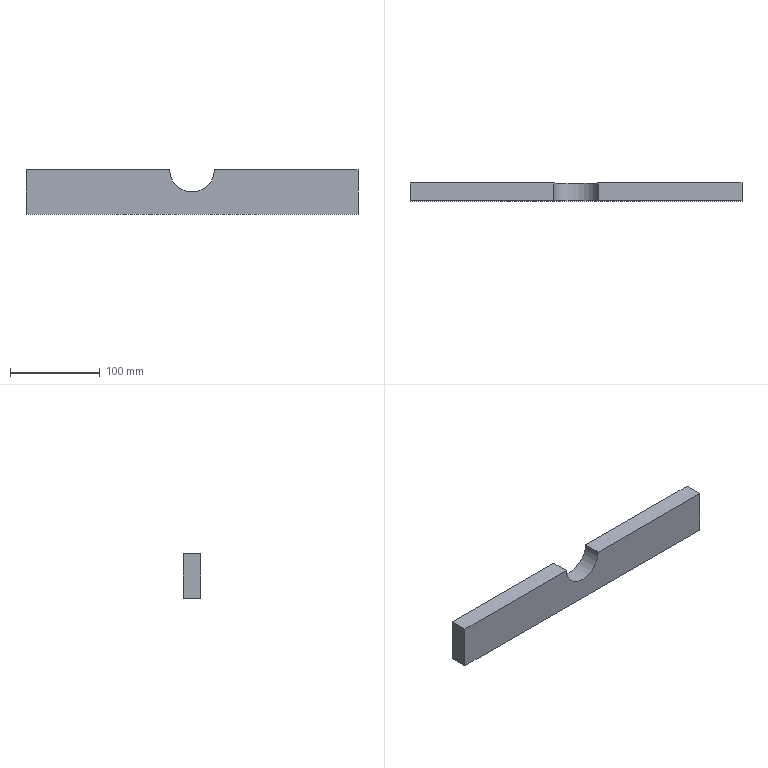Component | NX | TUTUCU_2 | 1 solid | 8 faces | box 370 x 20 x 50 mm | volume 350365 mm3 | plane 7 | cylinder 1 | commonest cylinder face diameters 50 x1
STEP:
#1=CARTESIAN_POINT('',(0.,0.,0.));
#2=DIRECTION('',(0.,0.,1.));
#3=DIRECTION('',(1.,0.,0.));
#4=AXIS2_PLACEMENT_3D('',#1,#2,#3);
#5=CARTESIAN_POINT('',(-1180.866,789.623,220.));
#6=VERTEX_POINT('',#5);
#7=CARTESIAN_POINT('',(-1180.866,769.623,220.));
#8=VERTEX_POINT('',#7);
#9=CARTESIAN_POINT('',(-1180.866,767.623,220.));
#10=DIRECTION('',(0.,-1.,0.));
#11=VECTOR('',#10,1.);
#12=LINE('',#9,#11);
#13=CARTESIAN_POINT('',(-970.866,789.623,220.));
#14=DIRECTION('',(0.,0.,-1.));
#15=DIRECTION('',(-1.,0.,0.));
#16=AXIS2_PLACEMENT_3D('',#13,#14,#15);
#17=PLANE('',#16);
#18=CARTESIAN_POINT('',(210.,-22.));
#19=DIRECTION('',(0.,-1.));
#20=VECTOR('',#19,1.);
#21=LINE('',#18,#20);
#22=(GEOMETRIC_REPRESENTATION_CONTEXT(2)PARAMETRIC_REPRESENTATION_CONTEXT()REPRESENTATION_CONTEXT('',''));
#23=DEFINITIONAL_REPRESENTATION('',(#21),#22);
#24=PCURVE('',#17,#23);
#25=CARTESIAN_POINT('',(-1155.866,767.623,220.));
#26=DIRECTION('',(0.,1.,0.));
#27=DIRECTION('',(0.,0.,1.));
#28=AXIS2_PLACEMENT_3D('',#25,#26,#27);
#29=CYLINDRICAL_SURFACE('',#28,25.);
#30=CARTESIAN_POINT('',(4.712,0.));
#31=DIRECTION('',(0.,-1.));
#32=VECTOR('',#31,1.);
#33=LINE('',#30,#32);
#34=(GEOMETRIC_REPRESENTATION_CONTEXT(2)PARAMETRIC_REPRESENTATION_CONTEXT()REPRESENTATION_CONTEXT('',''));
#35=DEFINITIONAL_REPRESENTATION('',(#33),#34);
#36=PCURVE('',#29,#35);
#37=SURFACE_CURVE('',#12,(#24,#36),.PCURVE_S1.);
#38=EDGE_CURVE('',#6,#8,#37,.T.);
#39=ORIENTED_EDGE('',*,*,#38,.F.);
#40=CARTESIAN_POINT('',(-1340.866,789.623,220.));
#41=VERTEX_POINT('',#40);
#42=CARTESIAN_POINT('',(-970.866,789.623,220.));
#43=DIRECTION('',(-1.,0.,0.));
#44=VECTOR('',#43,1.);
#45=LINE('',#42,#44);
#46=CARTESIAN_POINT('',(0.,0.));
#47=DIRECTION('',(1.,0.));
#48=VECTOR('',#47,1.);
#49=LINE('',#46,#48);
#50=(GEOMETRIC_REPRESENTATION_CONTEXT(2)PARAMETRIC_REPRESENTATION_CONTEXT()REPRESENTATION_CONTEXT('',''));
#51=DEFINITIONAL_REPRESENTATION('',(#49),#50);
#52=PCURVE('',#17,#51);
#53=CARTESIAN_POINT('',(-970.866,789.623,170.));
#54=DIRECTION('',(0.,-1.,-0.));
#55=DIRECTION('',(0.,0.,-1.));
#56=AXIS2_PLACEMENT_3D('',#53,#54,#55);
#57=PLANE('',#56);
#58=CARTESIAN_POINT('',(-50.,0.));
#59=DIRECTION('',(0.,-1.));
#60=VECTOR('',#59,1.);
#61=LINE('',#58,#60);
#62=(GEOMETRIC_REPRESENTATION_CONTEXT(2)PARAMETRIC_REPRESENTATION_CONTEXT()REPRESENTATION_CONTEXT('',''));
#63=DEFINITIONAL_REPRESENTATION('',(#61),#62);
#64=PCURVE('',#57,#63);
#65=SURFACE_CURVE('',#45,(#52,#64),.PCURVE_S1.);
#66=EDGE_CURVE('',#6,#41,#65,.T.);
#67=ORIENTED_EDGE('',*,*,#66,.T.);
#68=CARTESIAN_POINT('',(-1340.866,769.623,220.));
#69=VERTEX_POINT('',#68);
#70=CARTESIAN_POINT('',(-1340.866,789.623,220.));
#71=DIRECTION('',(0.,-1.,0.));
#72=VECTOR('',#71,1.);
#73=LINE('',#70,#72);
#74=CARTESIAN_POINT('',(370.,0.));
#75=DIRECTION('',(0.,-1.));
#76=VECTOR('',#75,1.);
#77=LINE('',#74,#76);
#78=(GEOMETRIC_REPRESENTATION_CONTEXT(2)PARAMETRIC_REPRESENTATION_CONTEXT()REPRESENTATION_CONTEXT('',''));
#79=DEFINITIONAL_REPRESENTATION('',(#77),#78);
#80=PCURVE('',#17,#79);
#81=CARTESIAN_POINT('',(-1340.866,769.623,170.));
#82=DIRECTION('',(1.,0.,0.));
#83=DIRECTION('',(0.,0.,-1.));
#84=AXIS2_PLACEMENT_3D('',#81,#82,#83);
#85=PLANE('',#84);
#86=CARTESIAN_POINT('',(-50.,20.));
#87=DIRECTION('',(0.,-1.));
#88=VECTOR('',#87,1.);
#89=LINE('',#86,#88);
#90=(GEOMETRIC_REPRESENTATION_CONTEXT(2)PARAMETRIC_REPRESENTATION_CONTEXT()REPRESENTATION_CONTEXT('',''));
#91=DEFINITIONAL_REPRESENTATION('',(#89),#90);
#92=PCURVE('',#85,#91);
#93=SURFACE_CURVE('',#73,(#80,#92),.PCURVE_S1.);
#94=EDGE_CURVE('',#41,#69,#93,.T.);
#95=ORIENTED_EDGE('',*,*,#94,.T.);
#96=CARTESIAN_POINT('',(-970.866,769.623,220.));
#97=DIRECTION('',(-1.,0.,0.));
#98=VECTOR('',#97,1.);
#99=LINE('',#96,#98);
#100=CARTESIAN_POINT('',(0.,-20.));
#101=DIRECTION('',(1.,0.));
#102=VECTOR('',#101,1.);
#103=LINE('',#100,#102);
#104=(GEOMETRIC_REPRESENTATION_CONTEXT(2)PARAMETRIC_REPRESENTATION_CONTEXT()REPRESENTATION_CONTEXT('',''));
#105=DEFINITIONAL_REPRESENTATION('',(#103),#104);
#106=PCURVE('',#17,#105);
#107=CARTESIAN_POINT('',(-970.866,769.623,220.));
#108=DIRECTION('',(0.,1.,0.));
#109=DIRECTION('',(0.,-0.,1.));
#110=AXIS2_PLACEMENT_3D('',#107,#108,#109);
#111=PLANE('',#110);
#112=CARTESIAN_POINT('',(0.,0.));
#113=DIRECTION('',(0.,-1.));
#114=VECTOR('',#113,1.);
#115=LINE('',#112,#114);
#116=(GEOMETRIC_REPRESENTATION_CONTEXT(2)PARAMETRIC_REPRESENTATION_CONTEXT()REPRESENTATION_CONTEXT('',''));
#117=DEFINITIONAL_REPRESENTATION('',(#115),#116);
#118=PCURVE('',#111,#117);
#119=SURFACE_CURVE('',#99,(#106,#118),.PCURVE_S1.);
#120=EDGE_CURVE('',#8,#69,#119,.T.);
#121=ORIENTED_EDGE('',*,*,#120,.F.);
#122=EDGE_LOOP('',(#39,#67,#95,#121));
#123=FACE_BOUND('',#122,.T.);
#124=ADVANCED_FACE('',(#123),#17,.F.);
#125=CARTESIAN_POINT('',(-1130.866,769.623,220.));
#126=VERTEX_POINT('',#125);
#127=CARTESIAN_POINT('',(-1130.866,789.623,220.));
#128=VERTEX_POINT('',#127);
#129=CARTESIAN_POINT('',(-1130.866,767.623,220.));
#130=DIRECTION('',(0.,1.,0.));
#131=VECTOR('',#130,1.);
#132=LINE('',#129,#131);
#133=CARTESIAN_POINT('',(-970.866,789.623,220.));
#134=DIRECTION('',(0.,0.,-1.));
#135=DIRECTION('',(-1.,0.,0.));
#136=AXIS2_PLACEMENT_3D('',#133,#134,#135);
#137=PLANE('',#136);
#138=CARTESIAN_POINT('',(160.,-22.));
#139=DIRECTION('',(0.,1.));
#140=VECTOR('',#139,1.);
#141=LINE('',#138,#140);
#142=(GEOMETRIC_REPRESENTATION_CONTEXT(2)PARAMETRIC_REPRESENTATION_CONTEXT()REPRESENTATION_CONTEXT('',''));
#143=DEFINITIONAL_REPRESENTATION('',(#141),#142);
#144=PCURVE('',#137,#143);
#145=CARTESIAN_POINT('',(1.571,0.));
#146=DIRECTION('',(0.,1.));
#147=VECTOR('',#146,1.);
#148=LINE('',#145,#147);
#149=(GEOMETRIC_REPRESENTATION_CONTEXT(2)PARAMETRIC_REPRESENTATION_CONTEXT()REPRESENTATION_CONTEXT('',''));
#150=DEFINITIONAL_REPRESENTATION('',(#148),#149);
#151=PCURVE('',#29,#150);
#152=SURFACE_CURVE('',#132,(#144,#151),.PCURVE_S1.);
#153=EDGE_CURVE('',#126,#128,#152,.T.);
#154=ORIENTED_EDGE('',*,*,#153,.F.);
#155=CARTESIAN_POINT('',(-970.866,769.623,220.));
#156=VERTEX_POINT('',#155);
#157=CARTESIAN_POINT('',(-970.866,769.623,220.));
#158=DIRECTION('',(-1.,0.,0.));
#159=VECTOR('',#158,1.);
#160=LINE('',#157,#159);
#161=CARTESIAN_POINT('',(0.,-20.));
#162=DIRECTION('',(1.,0.));
#163=VECTOR('',#162,1.);
#164=LINE('',#161,#163);
#165=(GEOMETRIC_REPRESENTATION_CONTEXT(2)PARAMETRIC_REPRESENTATION_CONTEXT()REPRESENTATION_CONTEXT('',''));
#166=DEFINITIONAL_REPRESENTATION('',(#164),#165);
#167=PCURVE('',#137,#166);
#168=CARTESIAN_POINT('',(0.,0.));
#169=DIRECTION('',(0.,-1.));
#170=VECTOR('',#169,1.);
#171=LINE('',#168,#170);
#172=(GEOMETRIC_REPRESENTATION_CONTEXT(2)PARAMETRIC_REPRESENTATION_CONTEXT()REPRESENTATION_CONTEXT('',''));
#173=DEFINITIONAL_REPRESENTATION('',(#171),#172);
#174=PCURVE('',#111,#173);
#175=SURFACE_CURVE('',#160,(#167,#174),.PCURVE_S1.);
#176=EDGE_CURVE('',#156,#126,#175,.T.);
#177=ORIENTED_EDGE('',*,*,#176,.F.);
#178=CARTESIAN_POINT('',(-970.866,789.623,220.));
#179=VERTEX_POINT('',#178);
#180=CARTESIAN_POINT('',(-970.866,789.623,220.));
#181=DIRECTION('',(0.,-1.,0.));
#182=VECTOR('',#181,1.);
#183=LINE('',#180,#182);
#184=CARTESIAN_POINT('',(0.,0.));
#185=DIRECTION('',(0.,-1.));
#186=VECTOR('',#185,1.);
#187=LINE('',#184,#186);
#188=(GEOMETRIC_REPRESENTATION_CONTEXT(2)PARAMETRIC_REPRESENTATION_CONTEXT()REPRESENTATION_CONTEXT('',''));
#189=DEFINITIONAL_REPRESENTATION('',(#187),#188);
#190=PCURVE('',#137,#189);
#191=CARTESIAN_POINT('',(-970.866,769.623,170.));
#192=DIRECTION('',(1.,0.,0.));
#193=DIRECTION('',(0.,0.,-1.));
#194=AXIS2_PLACEMENT_3D('',#191,#192,#193);
#195=PLANE('',#194);
#196=CARTESIAN_POINT('',(-50.,20.));
#197=DIRECTION('',(0.,-1.));
#198=VECTOR('',#197,1.);
#199=LINE('',#196,#198);
#200=(GEOMETRIC_REPRESENTATION_CONTEXT(2)PARAMETRIC_REPRESENTATION_CONTEXT()REPRESENTATION_CONTEXT('',''));
#201=DEFINITIONAL_REPRESENTATION('',(#199),#200);
#202=PCURVE('',#195,#201);
#203=SURFACE_CURVE('',#183,(#190,#202),.PCURVE_S1.);
#204=EDGE_CURVE('',#179,#156,#203,.T.);
#205=ORIENTED_EDGE('',*,*,#204,.F.);
#206=CARTESIAN_POINT('',(-970.866,789.623,220.));
#207=DIRECTION('',(-1.,0.,0.));
#208=VECTOR('',#207,1.);
#209=LINE('',#206,#208);
#210=CARTESIAN_POINT('',(0.,0.));
#211=DIRECTION('',(1.,0.));
#212=VECTOR('',#211,1.);
#213=LINE('',#210,#212);
#214=(GEOMETRIC_REPRESENTATION_CONTEXT(2)PARAMETRIC_REPRESENTATION_CONTEXT()REPRESENTATION_CONTEXT('',''));
#215=DEFINITIONAL_REPRESENTATION('',(#213),#214);
#216=PCURVE('',#137,#215);
#217=CARTESIAN_POINT('',(-50.,0.));
#218=DIRECTION('',(0.,-1.));
#219=VECTOR('',#218,1.);
#220=LINE('',#217,#219);
#221=(GEOMETRIC_REPRESENTATION_CONTEXT(2)PARAMETRIC_REPRESENTATION_CONTEXT()REPRESENTATION_CONTEXT('',''));
#222=DEFINITIONAL_REPRESENTATION('',(#220),#221);
#223=PCURVE('',#57,#222);
#224=SURFACE_CURVE('',#209,(#216,#223),.PCURVE_S1.);
#225=EDGE_CURVE('',#179,#128,#224,.T.);
#226=ORIENTED_EDGE('',*,*,#225,.T.);
#227=EDGE_LOOP('',(#154,#177,#205,#226));
#228=FACE_BOUND('',#227,.T.);
#229=ADVANCED_FACE('',(#228),#137,.F.);
#230=CARTESIAN_POINT('',(-1155.866,769.623,220.));
#231=DIRECTION('',(0.,-1.,-0.));
#232=DIRECTION('',(0.,-0.,1.));
#233=AXIS2_PLACEMENT_3D('',#230,#231,#232);
#234=CIRCLE('',#233,25.);
#235=CARTESIAN_POINT('',(25.,-185.));
#236=CARTESIAN_POINT('',(25.,-228.301));
#237=CARTESIAN_POINT('',(-12.5,-206.651));
#238=CARTESIAN_POINT('',(-50.,-185.));
#239=CARTESIAN_POINT('',(-12.5,-163.349));
#240=CARTESIAN_POINT('',(25.,-141.699));
#241=CARTESIAN_POINT('',(25.,-185.));
#242=(BOUNDED_CURVE()B_SPLINE_CURVE(2,(#235,#236,#237,#238,#239,#240,#241),.UNSPECIFIED.,.T.,.F.)B_SPLINE_CURVE_WITH_KNOTS((1,2,2,2,2,1),(-2.094,0.,2.094,4.189,6.283,8.378),.UNSPECIFIED.)CURVE()GEOMETRIC_REPRESENTATION_ITEM()RATIONAL_B_SPLINE_CURVE((1.,0.5,1.,0.5,1.,0.5,1.))REPRESENTATION_ITEM(''));
#243=(GEOMETRIC_REPRESENTATION_CONTEXT(2)PARAMETRIC_REPRESENTATION_CONTEXT()REPRESENTATION_CONTEXT('',''));
#244=DEFINITIONAL_REPRESENTATION('',(#242),#243);
#245=PCURVE('',#111,#244);
#246=CARTESIAN_POINT('',(6.283,2.));
#247=DIRECTION('',(-1.,0.));
#248=VECTOR('',#247,1.);
#249=LINE('',#246,#248);
#250=(GEOMETRIC_REPRESENTATION_CONTEXT(2)PARAMETRIC_REPRESENTATION_CONTEXT()REPRESENTATION_CONTEXT('',''));
#251=DEFINITIONAL_REPRESENTATION('',(#249),#250);
#252=PCURVE('',#29,#251);
#253=SURFACE_CURVE('',#234,(#245,#252),.PCURVE_S1.);
#254=EDGE_CURVE('',#8,#126,#253,.T.);
#255=ORIENTED_EDGE('',*,*,#254,.F.);
#256=ORIENTED_EDGE('',*,*,#120,.T.);
#257=CARTESIAN_POINT('',(-1340.866,769.623,170.));
#258=VERTEX_POINT('',#257);
#259=CARTESIAN_POINT('',(-1340.866,769.623,220.));
#260=DIRECTION('',(0.,0.,-1.));
#261=VECTOR('',#260,1.);
#262=LINE('',#259,#261);
#263=CARTESIAN_POINT('',(0.,-370.));
#264=DIRECTION('',(-1.,0.));
#265=VECTOR('',#264,1.);
#266=LINE('',#263,#265);
#267=(GEOMETRIC_REPRESENTATION_CONTEXT(2)PARAMETRIC_REPRESENTATION_CONTEXT()REPRESENTATION_CONTEXT('',''));
#268=DEFINITIONAL_REPRESENTATION('',(#266),#267);
#269=PCURVE('',#111,#268);
#270=CARTESIAN_POINT('',(-50.,0.));
#271=DIRECTION('',(1.,0.));
#272=VECTOR('',#271,1.);
#273=LINE('',#270,#272);
#274=(GEOMETRIC_REPRESENTATION_CONTEXT(2)PARAMETRIC_REPRESENTATION_CONTEXT()REPRESENTATION_CONTEXT('',''));
#275=DEFINITIONAL_REPRESENTATION('',(#273),#274);
#276=PCURVE('',#85,#275);
#277=SURFACE_CURVE('',#262,(#269,#276),.PCURVE_S1.);
#278=EDGE_CURVE('',#69,#258,#277,.T.);
#279=ORIENTED_EDGE('',*,*,#278,.T.);
#280=CARTESIAN_POINT('',(-970.866,769.623,170.));
#281=VERTEX_POINT('',#280);
#282=CARTESIAN_POINT('',(-970.866,769.623,170.));
#283=DIRECTION('',(-1.,0.,0.));
#284=VECTOR('',#283,1.);
#285=LINE('',#282,#284);
#286=CARTESIAN_POINT('',(-50.,0.));
#287=DIRECTION('',(0.,-1.));
#288=VECTOR('',#287,1.);
#289=LINE('',#286,#288);
#290=(GEOMETRIC_REPRESENTATION_CONTEXT(2)PARAMETRIC_REPRESENTATION_CONTEXT()REPRESENTATION_CONTEXT('',''));
#291=DEFINITIONAL_REPRESENTATION('',(#289),#290);
#292=PCURVE('',#111,#291);
#293=CARTESIAN_POINT('',(-970.866,769.623,170.));
#294=DIRECTION('',(0.,0.,1.));
#295=DIRECTION('',(1.,0.,0.));
#296=AXIS2_PLACEMENT_3D('',#293,#294,#295);
#297=PLANE('',#296);
#298=CARTESIAN_POINT('',(0.,0.));
#299=DIRECTION('',(-1.,0.));
#300=VECTOR('',#299,1.);
#301=LINE('',#298,#300);
#302=(GEOMETRIC_REPRESENTATION_CONTEXT(2)PARAMETRIC_REPRESENTATION_CONTEXT()REPRESENTATION_CONTEXT('',''));
#303=DEFINITIONAL_REPRESENTATION('',(#301),#302);
#304=PCURVE('',#297,#303);
#305=SURFACE_CURVE('',#285,(#292,#304),.PCURVE_S1.);
#306=EDGE_CURVE('',#281,#258,#305,.T.);
#307=ORIENTED_EDGE('',*,*,#306,.F.);
#308=CARTESIAN_POINT('',(-970.866,769.623,220.));
#309=DIRECTION('',(0.,0.,-1.));
#310=VECTOR('',#309,1.);
#311=LINE('',#308,#310);
#312=CARTESIAN_POINT('',(0.,0.));
#313=DIRECTION('',(-1.,0.));
#314=VECTOR('',#313,1.);
#315=LINE('',#312,#314);
#316=(GEOMETRIC_REPRESENTATION_CONTEXT(2)PARAMETRIC_REPRESENTATION_CONTEXT()REPRESENTATION_CONTEXT('',''));
#317=DEFINITIONAL_REPRESENTATION('',(#315),#316);
#318=PCURVE('',#111,#317);
#319=CARTESIAN_POINT('',(-50.,0.));
#320=DIRECTION('',(1.,0.));
#321=VECTOR('',#320,1.);
#322=LINE('',#319,#321);
#323=(GEOMETRIC_REPRESENTATION_CONTEXT(2)PARAMETRIC_REPRESENTATION_CONTEXT()REPRESENTATION_CONTEXT('',''));
#324=DEFINITIONAL_REPRESENTATION('',(#322),#323);
#325=PCURVE('',#195,#324);
#326=SURFACE_CURVE('',#311,(#318,#325),.PCURVE_S1.);
#327=EDGE_CURVE('',#156,#281,#326,.T.);
#328=ORIENTED_EDGE('',*,*,#327,.F.);
#329=ORIENTED_EDGE('',*,*,#176,.T.);
#330=EDGE_LOOP('',(#255,#256,#279,#307,#328,#329));
#331=FACE_BOUND('',#330,.T.);
#332=ADVANCED_FACE('',(#331),#111,.F.);
#333=CARTESIAN_POINT('',(-1155.866,789.623,220.));
#334=DIRECTION('',(0.,1.,0.));
#335=DIRECTION('',(-1.,0.,0.));
#336=AXIS2_PLACEMENT_3D('',#333,#334,#335);
#337=CIRCLE('',#336,25.);
#338=CARTESIAN_POINT('',(-50.,-210.));
#339=CARTESIAN_POINT('',(-93.301,-210.));
#340=CARTESIAN_POINT('',(-71.651,-172.5));
#341=CARTESIAN_POINT('',(-50.,-135.));
#342=CARTESIAN_POINT('',(-28.349,-172.5));
#343=CARTESIAN_POINT('',(-6.699,-210.));
#344=CARTESIAN_POINT('',(-50.,-210.));
#345=(BOUNDED_CURVE()B_SPLINE_CURVE(2,(#338,#339,#340,#341,#342,#343,#344),.UNSPECIFIED.,.T.,.F.)B_SPLINE_CURVE_WITH_KNOTS((1,2,2,2,2,1),(-2.094,0.,2.094,4.189,6.283,8.378),.UNSPECIFIED.)CURVE()GEOMETRIC_REPRESENTATION_ITEM()RATIONAL_B_SPLINE_CURVE((1.,0.5,1.,0.5,1.,0.5,1.))REPRESENTATION_ITEM(''));
#346=(GEOMETRIC_REPRESENTATION_CONTEXT(2)PARAMETRIC_REPRESENTATION_CONTEXT()REPRESENTATION_CONTEXT('',''));
#347=DEFINITIONAL_REPRESENTATION('',(#345),#346);
#348=PCURVE('',#57,#347);
#349=CARTESIAN_POINT('',(-1.571,22.));
#350=DIRECTION('',(1.,0.));
#351=VECTOR('',#350,1.);
#352=LINE('',#349,#351);
#353=(GEOMETRIC_REPRESENTATION_CONTEXT(2)PARAMETRIC_REPRESENTATION_CONTEXT()REPRESENTATION_CONTEXT('',''));
#354=DEFINITIONAL_REPRESENTATION('',(#352),#353);
#355=PCURVE('',#29,#354);
#356=SURFACE_CURVE('',#337,(#348,#355),.PCURVE_S1.);
#357=EDGE_CURVE('',#128,#6,#356,.T.);
#358=ORIENTED_EDGE('',*,*,#357,.F.);
#359=ORIENTED_EDGE('',*,*,#225,.F.);
#360=CARTESIAN_POINT('',(-970.866,789.623,170.));
#361=VERTEX_POINT('',#360);
#362=CARTESIAN_POINT('',(-970.866,789.623,170.));
#363=DIRECTION('',(0.,-0.,1.));
#364=VECTOR('',#363,1.);
#365=LINE('',#362,#364);
#366=CARTESIAN_POINT('',(0.,0.));
#367=DIRECTION('',(-1.,0.));
#368=VECTOR('',#367,1.);
#369=LINE('',#366,#368);
#370=(GEOMETRIC_REPRESENTATION_CONTEXT(2)PARAMETRIC_REPRESENTATION_CONTEXT()REPRESENTATION_CONTEXT('',''));
#371=DEFINITIONAL_REPRESENTATION('',(#369),#370);
#372=PCURVE('',#57,#371);
#373=CARTESIAN_POINT('',(0.,20.));
#374=DIRECTION('',(-1.,-0.));
#375=VECTOR('',#374,1.);
#376=LINE('',#373,#375);
#377=(GEOMETRIC_REPRESENTATION_CONTEXT(2)PARAMETRIC_REPRESENTATION_CONTEXT()REPRESENTATION_CONTEXT('',''));
#378=DEFINITIONAL_REPRESENTATION('',(#376),#377);
#379=PCURVE('',#195,#378);
#380=SURFACE_CURVE('',#365,(#372,#379),.PCURVE_S1.);
#381=EDGE_CURVE('',#361,#179,#380,.T.);
#382=ORIENTED_EDGE('',*,*,#381,.F.);
#383=CARTESIAN_POINT('',(-1340.866,789.623,170.));
#384=VERTEX_POINT('',#383);
#385=CARTESIAN_POINT('',(-970.866,789.623,170.));
#386=DIRECTION('',(-1.,0.,0.));
#387=VECTOR('',#386,1.);
#388=LINE('',#385,#387);
#389=CARTESIAN_POINT('',(0.,0.));
#390=DIRECTION('',(0.,-1.));
#391=VECTOR('',#390,1.);
#392=LINE('',#389,#391);
#393=(GEOMETRIC_REPRESENTATION_CONTEXT(2)PARAMETRIC_REPRESENTATION_CONTEXT()REPRESENTATION_CONTEXT('',''));
#394=DEFINITIONAL_REPRESENTATION('',(#392),#393);
#395=PCURVE('',#57,#394);
#396=CARTESIAN_POINT('',(0.,20.));
#397=DIRECTION('',(-1.,0.));
#398=VECTOR('',#397,1.);
#399=LINE('',#396,#398);
#400=(GEOMETRIC_REPRESENTATION_CONTEXT(2)PARAMETRIC_REPRESENTATION_CONTEXT()REPRESENTATION_CONTEXT('',''));
#401=DEFINITIONAL_REPRESENTATION('',(#399),#400);
#402=PCURVE('',#297,#401);
#403=SURFACE_CURVE('',#388,(#395,#402),.PCURVE_S1.);
#404=EDGE_CURVE('',#361,#384,#403,.T.);
#405=ORIENTED_EDGE('',*,*,#404,.T.);
#406=CARTESIAN_POINT('',(-1340.866,789.623,170.));
#407=DIRECTION('',(0.,-0.,1.));
#408=VECTOR('',#407,1.);
#409=LINE('',#406,#408);
#410=CARTESIAN_POINT('',(0.,-370.));
#411=DIRECTION('',(-1.,0.));
#412=VECTOR('',#411,1.);
#413=LINE('',#410,#412);
#414=(GEOMETRIC_REPRESENTATION_CONTEXT(2)PARAMETRIC_REPRESENTATION_CONTEXT()REPRESENTATION_CONTEXT('',''));
#415=DEFINITIONAL_REPRESENTATION('',(#413),#414);
#416=PCURVE('',#57,#415);
#417=CARTESIAN_POINT('',(0.,20.));
#418=DIRECTION('',(-1.,-0.));
#419=VECTOR('',#418,1.);
#420=LINE('',#417,#419);
#421=(GEOMETRIC_REPRESENTATION_CONTEXT(2)PARAMETRIC_REPRESENTATION_CONTEXT()REPRESENTATION_CONTEXT('',''));
#422=DEFINITIONAL_REPRESENTATION('',(#420),#421);
#423=PCURVE('',#85,#422);
#424=SURFACE_CURVE('',#409,(#416,#423),.PCURVE_S1.);
#425=EDGE_CURVE('',#384,#41,#424,.T.);
#426=ORIENTED_EDGE('',*,*,#425,.T.);
#427=ORIENTED_EDGE('',*,*,#66,.F.);
#428=EDGE_LOOP('',(#358,#359,#382,#405,#426,#427));
#429=FACE_BOUND('',#428,.T.);
#430=ADVANCED_FACE('',(#429),#57,.F.);
#431=CARTESIAN_POINT('',(-1340.866,769.623,170.));
#432=DIRECTION('',(0.,1.,0.));
#433=VECTOR('',#432,1.);
#434=LINE('',#431,#433);
#435=CARTESIAN_POINT('',(-370.,0.));
#436=DIRECTION('',(0.,1.));
#437=VECTOR('',#436,1.);
#438=LINE('',#435,#437);
#439=(GEOMETRIC_REPRESENTATION_CONTEXT(2)PARAMETRIC_REPRESENTATION_CONTEXT()REPRESENTATION_CONTEXT('',''));
#440=DEFINITIONAL_REPRESENTATION('',(#438),#439);
#441=PCURVE('',#297,#440);
#442=CARTESIAN_POINT('',(0.,0.));
#443=DIRECTION('',(0.,1.));
#444=VECTOR('',#443,1.);
#445=LINE('',#442,#444);
#446=(GEOMETRIC_REPRESENTATION_CONTEXT(2)PARAMETRIC_REPRESENTATION_CONTEXT()REPRESENTATION_CONTEXT('',''));
#447=DEFINITIONAL_REPRESENTATION('',(#445),#446);
#448=PCURVE('',#85,#447);
#449=SURFACE_CURVE('',#434,(#441,#448),.PCURVE_S1.);
#450=EDGE_CURVE('',#258,#384,#449,.T.);
#451=ORIENTED_EDGE('',*,*,#450,.T.);
#452=ORIENTED_EDGE('',*,*,#404,.F.);
#453=CARTESIAN_POINT('',(-970.866,769.623,170.));
#454=DIRECTION('',(0.,1.,0.));
#455=VECTOR('',#454,1.);
#456=LINE('',#453,#455);
#457=CARTESIAN_POINT('',(0.,0.));
#458=DIRECTION('',(0.,1.));
#459=VECTOR('',#458,1.);
#460=LINE('',#457,#459);
#461=(GEOMETRIC_REPRESENTATION_CONTEXT(2)PARAMETRIC_REPRESENTATION_CONTEXT()REPRESENTATION_CONTEXT('',''));
#462=DEFINITIONAL_REPRESENTATION('',(#460),#461);
#463=PCURVE('',#297,#462);
#464=CARTESIAN_POINT('',(0.,0.));
#465=DIRECTION('',(0.,1.));
#466=VECTOR('',#465,1.);
#467=LINE('',#464,#466);
#468=(GEOMETRIC_REPRESENTATION_CONTEXT(2)PARAMETRIC_REPRESENTATION_CONTEXT()REPRESENTATION_CONTEXT('',''));
#469=DEFINITIONAL_REPRESENTATION('',(#467),#468);
#470=PCURVE('',#195,#469);
#471=SURFACE_CURVE('',#456,(#463,#470),.PCURVE_S1.);
#472=EDGE_CURVE('',#281,#361,#471,.T.);
#473=ORIENTED_EDGE('',*,*,#472,.F.);
#474=ORIENTED_EDGE('',*,*,#306,.T.);
#475=EDGE_LOOP('',(#451,#452,#473,#474));
#476=FACE_BOUND('',#475,.T.);
#477=ADVANCED_FACE('',(#476),#297,.F.);
#478=ORIENTED_EDGE('',*,*,#327,.T.);
#479=ORIENTED_EDGE('',*,*,#472,.T.);
#480=ORIENTED_EDGE('',*,*,#381,.T.);
#481=ORIENTED_EDGE('',*,*,#204,.T.);
#482=EDGE_LOOP('',(#478,#479,#480,#481));
#483=FACE_BOUND('',#482,.T.);
#484=ADVANCED_FACE('',(#483),#195,.T.);
#485=ORIENTED_EDGE('',*,*,#278,.F.);
#486=ORIENTED_EDGE('',*,*,#94,.F.);
#487=ORIENTED_EDGE('',*,*,#425,.F.);
#488=ORIENTED_EDGE('',*,*,#450,.F.);
#489=EDGE_LOOP('',(#485,#486,#487,#488));
#490=FACE_BOUND('',#489,.T.);
#491=ADVANCED_FACE('',(#490),#85,.F.);
#492=ORIENTED_EDGE('',*,*,#357,.F.);
#493=ORIENTED_EDGE('',*,*,#153,.F.);
#494=ORIENTED_EDGE('',*,*,#254,.F.);
#495=ORIENTED_EDGE('',*,*,#38,.F.);
#496=EDGE_LOOP('',(#492,#493,#494,#495));
#497=FACE_BOUND('',#496,.F.);
#498=ADVANCED_FACE('',(#497),#29,.F.);
#499=CLOSED_SHELL('',(#124,#229,#332,#430,#477,#484,#491,#498));
#500=MANIFOLD_SOLID_BREP('',#499);
#501=(LENGTH_UNIT()NAMED_UNIT(*)SI_UNIT(.MILLI.,.METRE.));
#502=UNCERTAINTY_MEASURE_WITH_UNIT(LENGTH_MEASURE(0.0000001),#501,'','');
#503=(NAMED_UNIT(*)PLANE_ANGLE_UNIT()SI_UNIT($,.RADIAN.));
#504=(NAMED_UNIT(*)SI_UNIT($,.STERADIAN.)SOLID_ANGLE_UNIT());
#505=(GEOMETRIC_REPRESENTATION_CONTEXT(3)GLOBAL_UNCERTAINTY_ASSIGNED_CONTEXT((#502))GLOBAL_UNIT_ASSIGNED_CONTEXT((#501,#503,#504))REPRESENTATION_CONTEXT('',''));
#506=ADVANCED_BREP_SHAPE_REPRESENTATION('',(#4,#500),#505);